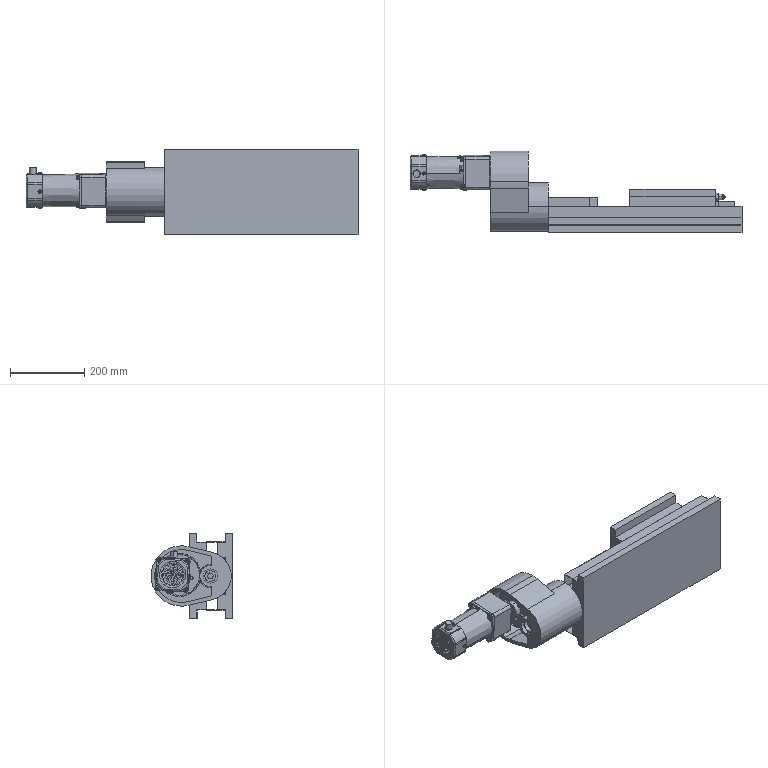Assembly | SolidWorks | mm | 44 component files | 283 solids | 3099 faces | box 892.1 x 219.71 x 230 mm | volume 9182823 mm3 | cylinder 1035 | sphere 848 | plane 712 | spline 244 | cone 148 | torus 112 | commonest cylinder face diameters 115.5 x76 108.75 x75 2 x53 20 x52 15 x47 39 x38 50.25 x36 57 x36
Bill of materials:
BallScrew | 1 |  | Long, slender solid rod with stepped smaller-diameter sections at both ends and a band of closely spaced grooves partway along its length.
BearingHousing | 1 |  | Two separate prismatic bodies: a thin rectangular block with a round through-hole and a stepped notch along one lower edge, beside a solid rectangular block with no visible features.
ConnectingFlange | 2 |  | Long, constant-section, thin-walled bent profile. Its cross-section has a flat web, offset parallel flanges, and short return lips with small inside bend radii.
ConnectingSeat | 1 |  | Rectangular block with a large round through-bore along its length. One side has a wider flange-like section, so the end profile is T-shaped.
CopperGasket | 1 |  | Two separate thin flat plates: a rectangular plate with four small holes near its corners, and a long narrow strip with no visible holes.
CountersunkScrewM5X20 | 6 |  | Stepped cylindrical pin with a larger cylindrical head, a recessed drive socket in the head end face, and a smaller plain shank with a chamfered tip.
CountersunkScrewM8x4 | 4 |  | Stepped cylindrical pin with a larger cylindrical head and a smaller plain shank with a chamfered end.
CouplingSleeve | 1 |  | Plain cylindrical sleeve or tube with a smooth outside and a round bore with one rectangular keyway notch running along the bore.
DeepGrooveBallBearing16002 | 5 |  | Flat annular assembly with an outer ring, a wide inner ring around a central bore, and a circle of spherical balls between them, resembling a ball bearing.
DeepGrooveBallBearing6204 | 1 |  | Thin-section annular assembly with a large bore, an inner and an outer ring, and a circle of spherical balls between them, resembling a thin-section ball bearing.
EndCap | 1 |  | Bracket-like block with a flat mounting flange holding four through-holes and a body with a large circular bore. The bore has an internal shoulder and four rectangular relief notches around it.
Gearbox | 1 |  | Solid stepped body with a cam- or pear-shaped lobe section and an adjacent narrower section. An off-center round through-hole sits near the smaller rounded end.
GearboxLargeGear | 1 |  | Large spur gear with straight teeth around the rim, a central bore, six round lightening holes evenly spaced around the bore, and a cylindrical hub boss on one face.
GearboxSmallGear | 1 |  | Small spur gear (pinion) with straight teeth, a central round through-bore, and a cylindrical hub on one side. The hub is about as long as the toothed face is wide.
GearShaft | 1 |  | Long, slender solid round shaft with a short rectangular slot or flat cut near each end. The two cuts appear to be on different sides of the shaft.
HexSocketScrewM6X15 | 1 |  | Socket-head-cap-screw-like part: a cylindrical head with a hexagonal socket recess, and a plain cylindrical shank with a chamfered tip.
NutSeat | 1 |  | Solid rectangular block with one round hole in a smaller end face. The hole sits off-centre on that face.
OilCup | 1 |  | Turned stepped part. It has a short cylindrical collar, a hexagonal flange, a cylindrical body, a smaller chamfered step, and ends in a small cylindrical pin with a conical point.
OriginalWasher | 2 |  | Thin-walled plain ring: a short hollow cylinder with a large bore relative to its outside diameter.
ParallelKey5x5x25 | 1 |  | Solid prism with flat parallel faces and rounded (obround) ends, shaped like a rectangular bar with semicircular ends.
RoundNut | 2 |  | Thick flat ring or washer with a central round hole, flat parallel faces and a plain cylindrical outer edge.
RoundNutLockingWasher15 | 2 |  | Thin flat washer-like disc with a central hole. The outer edge is bevelled on one face, giving a conical outer rim.
SealingAnvil | 1 |  | Flat plate of uniform thickness with a stepped outline: a tall narrow strip along one side joined to a wider, shorter rectangular tab. The tab has one round through-hole.
SealingFelt | 1 |  | Washer-like ring with a central round hole. Both faces are chamfered or bevelled at the outer edge, giving a double-tapered side profile.
ShaftRetainingRing | 1 |  | Thin flat annular ring (washer-like disc) with one concentric central through hole.
StepperMotor | 1 |  | Elongated motor-like body: a cylindrical main housing between a rounded rear end cap and a square front housing, with a cylindrical output shaft sticking out of the centre of the square front face.
WorkPlatform | 1 |  | Square flat plate with two parallel raised rails along opposite edges of one face, and six small through holes in two columns of three in the centre area.
X-AxisSupportBase | 1 |  | Long rectangular flat plate. One face is plain; the other has two raised outer ribs and a wider, slightly lower central raised strip, separated from the ribs by narrow grooves, all running along the length.
Mates:
1. parallel | X-AxisSupportBase-1 face at (0, 40, 90.896) dir (0, 0, 1) | ConnectingFlange-3 face at (-277, 70, 90.896) dir (0, 0, -1)
2. parallel | X-AxisSupportBase-1 face at (-277, 20, 115) dir (-1, 0, 0) | ConnectingFlange-3 face at (-277, 70, 91.632) dir (-1, 0, 0)
3. coincident | X-AxisSupportBase-1 face at (-277, 20, 115) dir (-1, 0, 0) | ConnectingFlange-3 face at (-277, 70, 48.661) dir (-1, 0, 0)
4. coincident | X-AxisSupportBase-1 face at (0, 20, 0) dir (0, 1, 0) | ConnectingFlange-3 face at (0, 20, 0) dir (0, -1, 0)
5. coincident | X-AxisSupportBase-1 face at (503, 0, 49.398) dir (0, 0, -1) | ConnectingFlange-3 face at (0, 20, 49.398) dir (0, 0, 1)
6. parallel | X-AxisSupportBase-1 face at (0, 0, 0) dir (0, -1, 0) | WorkPlatform-1 face at (56.772, 116.74, 0) dir (0, 1, 0)
7. parallel | X-AxisSupportBase-1 face at (-277, 20, 115) dir (0, 0, 1) | WorkPlatform-1 face at (171.772, 116.74, 115) dir (0, 0, 1)
8. coincident | X-AxisSupportBase-1 face at (0, 20, 0) dir (0, 1, 0) | ConnectingSeat-1 face at (-166, 20, 46.072) dir (0, -1, 0)
9. coincident | X-AxisSupportBase-1 face at (-277, 20, 115) dir (-1, 0, 0) | ConnectingSeat-1 face at (-277, 40, 0) dir (-1, 0, 0)
10. coincident | ConnectingSeat-1 face at (-277, 40, 0) dir (-1, 0, 0) | Gearbox-1 face at (-277, 69.2, 0) dir (1, 0, 0)
11. concentric | Gearbox-1 face at (-302, 60.219, 0) dir (1, 0, 0) r 25.57 | GearboxSmallGear-1 face at (-323.574, 60.219, 0) dir (-1, 0, 0) r 7.5
12. coincident | Gearbox-1 plane at (-277, 0, 0) dir (0, 0, -1) | assembly plane at (0, 0, 0) dir (0, 0, 1)
13. concentric | BallScrew-1 face at (263, 60.219, 0) dir (1, 0, 0) r 7.5 | BearingHousing-1 face at (194.019, 60.219, 0) dir (-1, 0, 0) r 10.5
14. concentric | BallScrew-1 face at (263, 60.219, 0) dir (-1, 0, 0) r 10 | NutSeat-1 face at (-31.284, 60.219, 0) dir (1, 0, 0) r 10
15. coincident | BallScrew-1 sketch segment at (103, 60.219, 0) dir (1, 0, 0) r 10 | NutSeat-1 sketch segment at (103, 60.219, 0) dir (1, 0, 0) r 10
16. concentric | ConnectingSeat-1 face at (-281, 60.219, 0) dir (1, 0, 0) r 25.57 | DeepGrooveBallBearing16002-1 face at (-186, 60.219, 0) dir (-1, 0, 0) r 23.5
17. coincident | ConnectingSeat-1 face at (-166, 40, 0) dir (1, 0, 0) | DeepGrooveBallBearing16002-2 face at (-166, 82.472, 6.559) dir (1, 0, 0)
18. concentric | BallScrew-1 face at (-250, 60.219, 0) dir (1, 0, 0) r 6.215 | CouplingSleeve-1 face at (-286.5, 60.219, 0) dir (1, 0, 0) r 8.58
19. distance | GearShaft-1 face at (-277, 60.219, 0) dir (1, 0, 0) | BallScrew-1 face at (-272, 60.219, 0) dir (-1, 0, 0)
20. coincident | GearboxSmallGear-1 face at (-413, 60.219, 0) dir (-1, 0, 0) | GearShaft-1 face at (-413, 60.219, 0) dir (-1, 0, 0)
21. coincident | GearShaft-1 face at (-282, 56.727, -0.07861) dir (0, 0.7323, 0.681) | ParallelKey5x5x25-1 face at (-14.748, 51.96, 5.047) dir (0, -0.7323, -0.681)
22. coincident | BallScrew-1 face at (-265, 56.727, -0.07861) dir (0, 0.7323, 0.681) | ParallelKey5x5x25-1 face at (-14.748, 51.96, 5.047) dir (0, -0.7323, -0.681)
23. coincident | GearShaft-1 face at (-282, 56.727, -0.07861) dir (0, -0.681, 0.7323) | ParallelKey5x5x25-1 edge at (-280.428, 56.727, -0.07861) dir (1, 0, 0)
24. coincident | BallScrew-1 face at (-265, 56.727, -0.07861) dir (0, -0.681, 0.7323) | ParallelKey5x5x25-1 edge at (-280.428, 56.727, -0.07861) dir (1, 0, 0)
25. tangent | GearShaft-1 face at (-282, 101.228, -44.098) dir (1, 0, 0) | ParallelKey5x5x25-1 face at (-279.134, 58.6, 1.663) dir (0, -0.681, 0.7323) r 2.866
26. concentric | BallScrew-1 face at (-250, 60.219, 0) dir (1, 0, 0) r 6.215 | Gearbox-1 face at (-292, 60.219, 0) dir (1, 0, 0) r 18.564
27. concentric | Gearbox-1 face at (-398.993, 60.219, 0) dir (-1, 0, 0) r 15 | GearShaft-1 edge at (-413, 60.219, 0) dir (-1, 0, 0) r 7.5
28. coincident | BallScrew-1 edge at (-249.5, 60.219, 0) dir (1, 0, 0) r 6.215 | CouplingSleeve-1 face at (-249.5, 60.219, 0) dir (1, 0, 0)
29. concentric | BallScrew-1 face at (263, 60.219, 0) dir (-1, 0, 0) r 10 | RoundNutLockingWasher15-1 edge at (-186, 60.219, 0) dir (-1, 0, 0) r 10.006
30. concentric | BallScrew-1 face at (263, 60.219, 0) dir (-1, 0, 0) r 10 | RoundNut-1 face at (-196.75, 60.219, 0) dir (1, 0, 0) r 19.5
31. coincident | RoundNut-1 edge at (-187.75, 60.219, 0) dir (-1, 0, 0) r 19.5 | RoundNutLockingWasher15-1 edge at (-187.75, 60.219, 0) dir (-1, 0, 0) r 19.5
32. coincident | DeepGrooveBallBearing16002-1 face at (-186, 52.87, -16.212) dir (-1, 0, 0) | RoundNutLockingWasher15-1 face at (-186, 80.498, 0) dir (1, 0, 0)
33. coincident | DeepGrooveBallBearing16002-1 face at (-179, 52.168, -17.76) dir (1, 0, 0) | OriginalWasher-1 face at (-179, 59.486, -0.1318) dir (-1, 0, 0)
34. coincident | DeepGrooveBallBearing16002-2 face at (-173, 77.293, 5.033) dir (-1, 0, 0) | OriginalWasher-1 face at (-173, 59.486, -0.1318) dir (1, 0, 0)
35. concentric | BallScrew-1 face at (263, 60.219, 0) dir (-1, 0, 0) r 10 | OriginalWasher-1 face at (-176, 60.219, 0) dir (1, 0, 0) r 16.311
36. coincident | Gearbox-1 face at (-331, 60.219, 0) dir (-1, 0, 0) | DeepGrooveBallBearing16002-4 face at (-331, 83.419, 0) dir (-1, 0, 0)
37. concentric | BallScrew-1 face at (263, 60.219, 0) dir (-1, 0, 0) r 10 | SealingAnvil-1 face at (-146, 60.219, 0) dir (-1, 0, 0) r 10
38. parallel | X-AxisSupportBase-1 face at (0, 20, 0) dir (0, 1, 0) | SealingAnvil-1 face at (-146, 39.822, -46.072) dir (0, 1, 0)
39. coincident | X-AxisSupportBase-1 face at (0, 20, 0) dir (0, 1, 0) | SealingAnvil-1 edge at (-166, 20, 45.25) dir (0, 0, -1)
40. coincident | ConnectingSeat-1 face at (-166, 40, 0) dir (1, 0, 0) | SealingAnvil-1 face at (-166, 0, 0) dir (-1, 0, 0)
41. concentric | BallScrew-1 face at (263, 60.219, 0) dir (-1, 0, 0) r 10 | DeepGrooveBallBearing16002-5 face at (208.13, 60.219, 0) dir (-1, 0, 0) r 11.01
42. concentric | BallScrew-1 face at (263, 60.219, 0) dir (1, 0, 0) r 7.5 | DeepGrooveBallBearing16002-6 face at (221.13, 60.219, 0) dir (-1, 0, 0) r 11.01
43. concentric | BallScrew-1 face at (263, 60.219, 0) dir (1, 0, 0) r 7.5 | OriginalWasher-2 face at (160.784, 60.219, 0) dir (1, 0, 0) r 19.557
44. coincident | DeepGrooveBallBearing16002-5 face at (157.784, 66.274, 18.536) dir (1, 0, 0) | OriginalWasher-2 face at (157.784, 59.486, -0.1289) dir (-1, 0, 0)
45. coincident | DeepGrooveBallBearing16002-6 face at (163.784, 75.449, 9.213) dir (-1, 0, 0) | OriginalWasher-2 face at (163.784, 59.486, -0.1289) dir (1, 0, 0)
46. coincident | DeepGrooveBallBearing16002-6 face at (170.784, 76.904, 10.093) dir (1, 0, 0) | RoundNutLockingWasher15-2 face at (170.784, 63.673, 19.982) dir (-1, 0, 0)
47. concentric | RoundNutLockingWasher15-2 edge at (172.384, 60.219, 0) dir (1, 0, 0) r 10.006 | RoundNut-2 face at (172.534, 60.219, 0) dir (1, 0, 0) r 10
48. coincident | RoundNutLockingWasher15-2 face at (172.534, 60.219, 0) dir (-1, 0, 0) r 1554.999 | RoundNut-2 edge at (172.534, 60.219, 0) dir (-1, 0, 0) r 19.5
49. concentric | Gearbox-1 face at (-425, 60.219, 0) dir (-1, 0, 0) r 19.092 | DeepGrooveBallBearing6204-2 face at (-413, 60.219, 0) dir (-1, 0, 0) r 15
50. coincident | Gearbox-1 face at (-406, 60.219, 0) dir (1, 0, 0) | DeepGrooveBallBearing6204-2 face at (-406, 80.67, -3.201) dir (1, 0, 0)
51. parallel | GearboxSmallGear-1 face at (-396, 57.853, 1.33) dir (0, 0.8717, -0.4901) | GearShaft-1 face at (-388.806, 48.864, -14.657) dir (0, 0.8717, -0.4901)
52. coincident | GearboxSmallGear-1 face at (-366, 60.219, 0) dir (1, 0, 0) | ShaftRetainingRing-1 edge at (-366, 60.219, 0) dir (1, 0, 0) r 15.026
53. coincident | GearboxSmallGear-1 face at (-413, 60.219, 0) dir (-1, 0, 0) | DeepGrooveBallBearing6204-2 edge at (-413, 60.219, 0) dir (-1, 0, 0) r 15.3
54. parallel | GearboxSmallGear-1 face at (-413, 60.219, 0) dir (-1, 0, 0) | GearboxLargeGear-4 face at (-410, 143.601, 2.729) dir (-1, 0, 0)
55. concentric | StepperMotor-2 face at (-426.5, 143.601, 2.729) dir (1, 0, 0) r 7.5 | GearboxLargeGear-4 face at (-318, 143.601, 2.729) dir (-1, 0, 0) r 14.069
56. coincident | Gearbox-1 face at (-434, 138.635, 0) dir (-1, 0, 0) | StepperMotor-2 face at (-434, 161.576, 3.68) dir (1, 0, 0)
57. coincident | GearboxLargeGear-4 face at (-376, 120.86, 26.56) dir (1, 0, 0) | CountersunkScrewM5X20-1 edge at (-376, 120.86, 26.56) dir (1, 0, 0) r 7.5
58. concentric | GearboxLargeGear-4 face at (-376, 120.86, 26.56) dir (1, 0, 0) r 7.5 | CountersunkScrewM5X20-1 face at (-362, 120.86, 26.56) dir (-1, 0, 0) r 7.5
59. coincident | WorkPlatform-1 face at (56.772, 96.74, 0) dir (0, -1, 0) | CopperGasket-1 face at (-3, 96.74, 0) dir (0, 1, 0)
60. concentric | WorkPlatform-1 face at (86.571, 106.74, -20.473) dir (0, 1, 0) r 4.017 | CountersunkScrewM8x4-2 face at (86.571, 87.74, -20.473) dir (0, 1, 0) r 2.271
61. concentric | WorkPlatform-1 face at (86.571, 58.74, 20.473) dir (0, 1, 0) r 2.271 | CountersunkScrewM8x4-4 face at (86.571, 87.74, 20.473) dir (0, 1, 0) r 2.271
62. concentric | WorkPlatform-1 face at (26.973, 58.74, 20.473) dir (0, 1, 0) r 2.271 | CountersunkScrewM8x4-3 face at (26.973, 87.74, 20.473) dir (0, 1, 0) r 2.271
63. coincident | GearboxSmallGear-1 face at (-396, 60.219, 0) dir (-1, 0, 0) | GearboxLargeGear-4 face at (-396, 143.601, 2.729) dir (-1, 0, 0)
64. gear | GearboxSmallGear-1 sketch segment at (-396, 60.219, 0) dir (-1, 0, 0) r 26.846 | GearboxLargeGear-4 sketch segment at (-396, 143.601, 2.729) dir (-1, 0, 0) r 56.581
65. coincident | BearingHousing-1 edge at (178.784, 84.114, -27.5) dir (0, 0, 1) | EndCap-2 face at (178.784, 77.114, 0) dir (1, 0, 0)
66. coincident | BearingHousing-1 face at (-54.961, 84.114, 27.5) dir (0, 1, 0) | EndCap-2 face at (158.784, 84.114, -27.5) dir (0, 1, 0)
67. coincident | BearingHousing-1 face at (-54.961, 85.587, 27.5) dir (0, 0, 1) | EndCap-2 face at (158.784, 84.114, 27.5) dir (0, 0, 1)
68. concentric | X-AxisSupportBase-1 face at (157.679, 36, 37.292) dir (0, -1, 0) r 2.542 | EndCap-2 face at (157.679, 32.078, 37.292) dir (0, 1, 0) r 2.542
69. concentric | BallScrew-1 face at (263, 60.219, 0) dir (-1, 0, 0) r 10 | RoundNut-2 face at (172.534, 60.219, 0) dir (1, 0, 0) r 19.5
70. concentric | GearShaft-1 face at (-277, 60.219, 0) dir (-1, 0, 0) r 7.5 | ShaftRetainingRing-1 face at (-363, 60.219, 0) dir (-1, 0, 0) r 7.5
71. parallel | CouplingSleeve-1 face at (-286.5, 55.015, 1.689) dir (0, 0.7323, 0.681) | ParallelKey5x5x25-1 face at (-14.748, 55.784, 8.603) dir (0, 0.7323, 0.681)
72. coincident | EndCap-2 face at (150.784, 85.587, 21.161) dir (-1, 0, 0) | DeepGrooveBallBearing16002-5 face at (150.784, 67.423, 22.053) dir (-1, 0, 0)